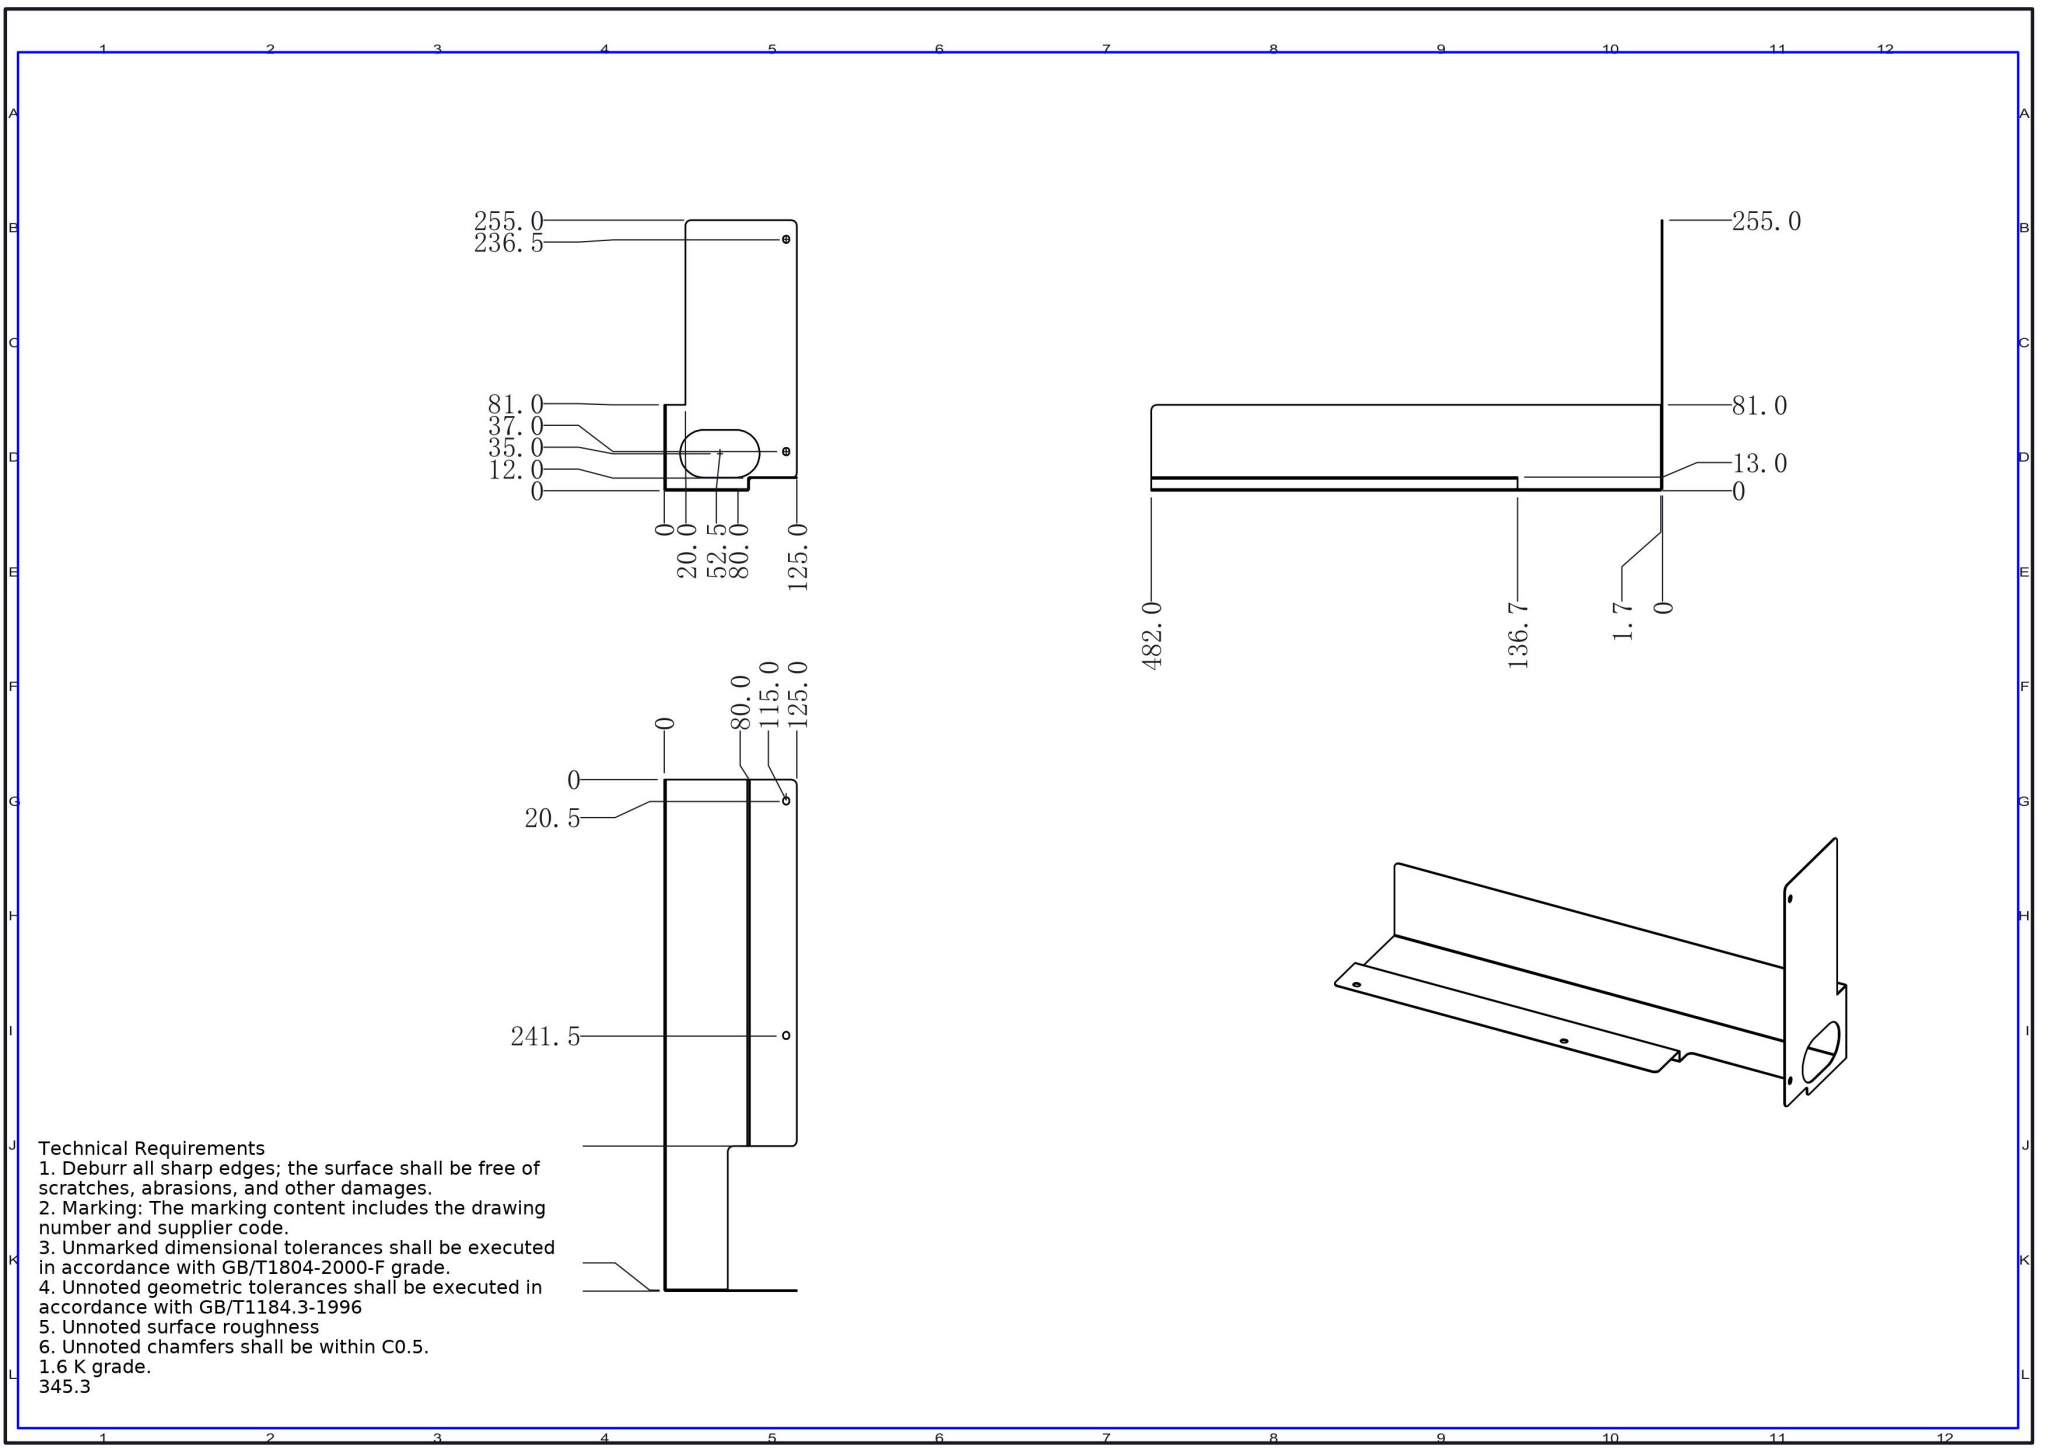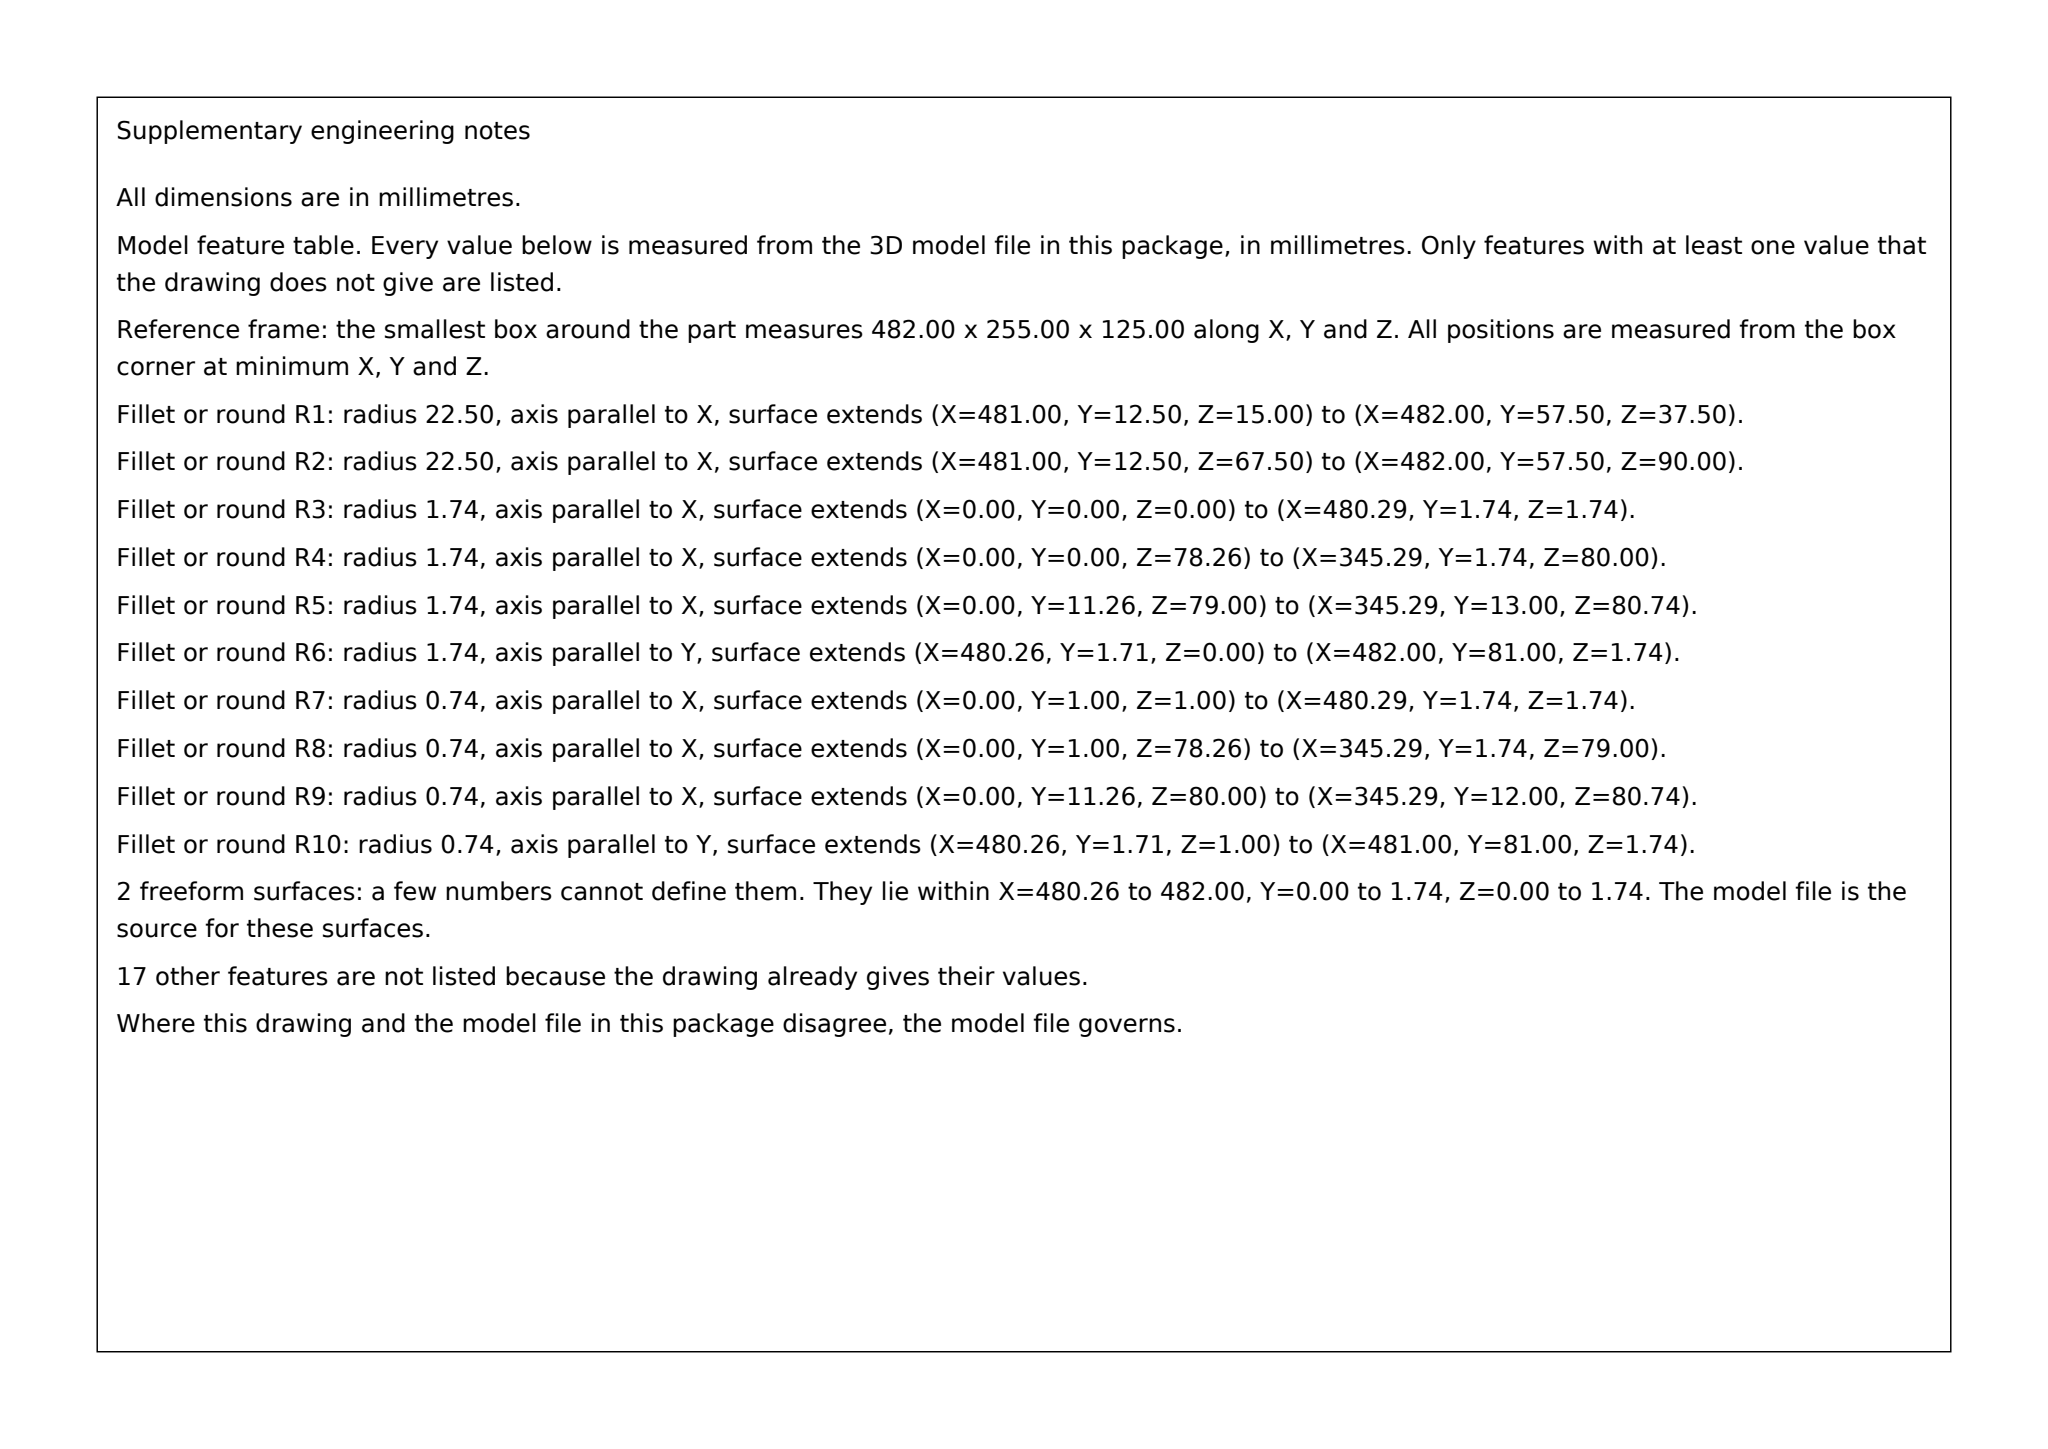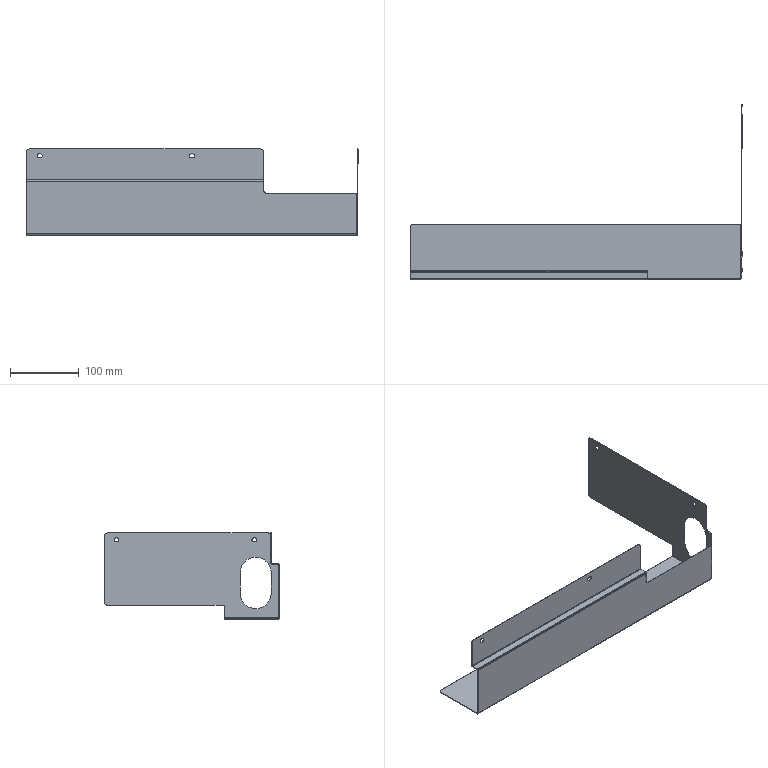Part | SolidWorks | mm | 1 solid | 74 faces | box 482 x 255 x 125 mm | volume 117835 mm3 | plane 44 | cylinder 28 | spline 2 | commonest cylinder face diameters 6 x10 10 x7 3.473 x4 1.473 x4 45 x3